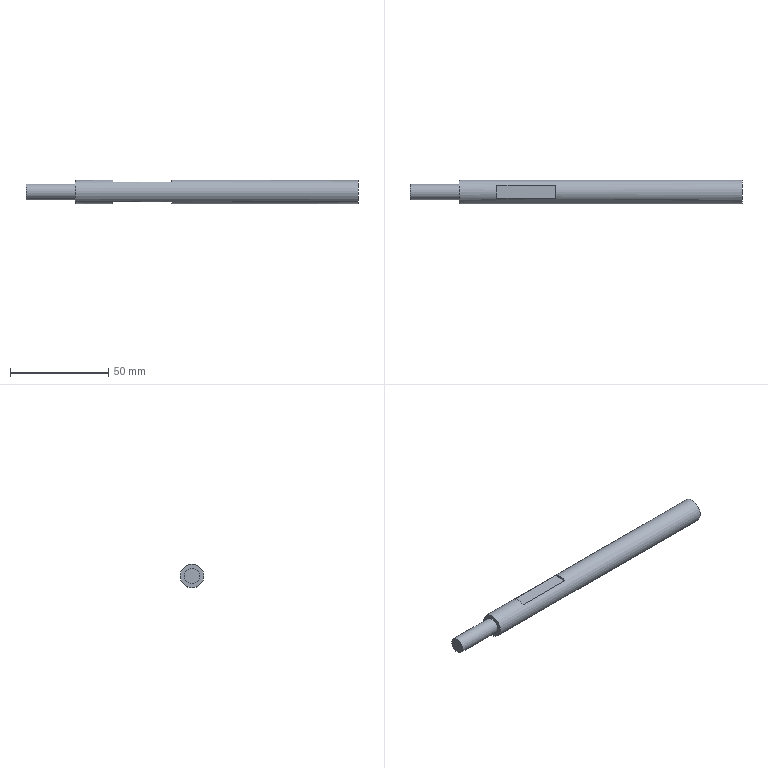Component | NX | LOCKING_SHAFT | 1 solid | 11 faces | box 169 x 12 x 12 mm | volume 17273 mm3 | plane 9 | cylinder 2 | commonest cylinder face diameters 12 x1 8 x1
STEP:
#1=CARTESIAN_POINT('',(0.,0.,0.));
#2=DIRECTION('',(0.,0.,1.));
#3=DIRECTION('',(1.,0.,0.));
#4=AXIS2_PLACEMENT_3D('',#1,#2,#3);
#5=CARTESIAN_POINT('',(-23.708,70.304,196.845));
#6=VERTEX_POINT('',#5);
#7=CARTESIAN_POINT('',(-23.708,76.937,196.845));
#8=VERTEX_POINT('',#7);
#9=CARTESIAN_POINT('',(-23.708,73.621,201.845));
#10=DIRECTION('',(1.,0.,0.));
#11=DIRECTION('',(0.,0.,1.));
#12=AXIS2_PLACEMENT_3D('',#9,#10,#11);
#13=CIRCLE('',#12,6.);
#14=CARTESIAN_POINT('',(-23.708,73.621,201.845));
#15=DIRECTION('',(-1.,0.,0.));
#16=DIRECTION('',(0.,0.,1.));
#17=AXIS2_PLACEMENT_3D('',#14,#15,#16);
#18=PLANE('',#17);
#19=CARTESIAN_POINT('',(6.,0.));
#20=CARTESIAN_POINT('',(6.,-10.392));
#21=CARTESIAN_POINT('',(-3.,-5.196));
#22=CARTESIAN_POINT('',(-12.,-0.));
#23=CARTESIAN_POINT('',(-3.,5.196));
#24=CARTESIAN_POINT('',(6.,10.392));
#25=CARTESIAN_POINT('',(6.,0.));
#26=(BOUNDED_CURVE()B_SPLINE_CURVE(2,(#19,#20,#21,#22,#23,#24,#25),.UNSPECIFIED.,.T.,.F.)B_SPLINE_CURVE_WITH_KNOTS((1,2,2,2,2,1),(-2.094,0.,2.094,4.189,6.283,8.378),.UNSPECIFIED.)CURVE()GEOMETRIC_REPRESENTATION_ITEM()RATIONAL_B_SPLINE_CURVE((1.,0.5,1.,0.5,1.,0.5,1.))REPRESENTATION_ITEM(''));
#27=(GEOMETRIC_REPRESENTATION_CONTEXT(2)PARAMETRIC_REPRESENTATION_CONTEXT()REPRESENTATION_CONTEXT('',''));
#28=DEFINITIONAL_REPRESENTATION('',(#26),#27);
#29=PCURVE('',#18,#28);
#30=CARTESIAN_POINT('',(71.092,73.621,201.845));
#31=DIRECTION('',(-1.,0.,0.));
#32=DIRECTION('',(0.,0.,1.));
#33=AXIS2_PLACEMENT_3D('',#30,#31,#32);
#34=CYLINDRICAL_SURFACE('',#33,6.);
#35=CARTESIAN_POINT('',(6.283,94.8));
#36=DIRECTION('',(-1.,0.));
#37=VECTOR('',#36,1.);
#38=LINE('',#35,#37);
#39=(GEOMETRIC_REPRESENTATION_CONTEXT(2)PARAMETRIC_REPRESENTATION_CONTEXT()REPRESENTATION_CONTEXT('',''));
#40=DEFINITIONAL_REPRESENTATION('',(#38),#39);
#41=PCURVE('',#34,#40);
#42=SURFACE_CURVE('',#13,(#29,#41),.PCURVE_S1.);
#43=EDGE_CURVE('',#6,#8,#42,.T.);
#44=ORIENTED_EDGE('',*,*,#43,.F.);
#45=CARTESIAN_POINT('',(-23.708,73.621,196.845));
#46=DIRECTION('',(0.,1.,0.));
#47=VECTOR('',#46,1.);
#48=LINE('',#45,#47);
#49=CARTESIAN_POINT('',(-5.,0.));
#50=DIRECTION('',(0.,1.));
#51=VECTOR('',#50,1.);
#52=LINE('',#49,#51);
#53=(GEOMETRIC_REPRESENTATION_CONTEXT(2)PARAMETRIC_REPRESENTATION_CONTEXT()REPRESENTATION_CONTEXT('',''));
#54=DEFINITIONAL_REPRESENTATION('',(#52),#53);
#55=PCURVE('',#18,#54);
#56=CARTESIAN_POINT('',(71.092,73.621,196.845));
#57=DIRECTION('',(0.,0.,-1.));
#58=DIRECTION('',(-1.,0.,0.));
#59=AXIS2_PLACEMENT_3D('',#56,#57,#58);
#60=PLANE('',#59);
#61=CARTESIAN_POINT('',(94.8,0.));
#62=DIRECTION('',(0.,1.));
#63=VECTOR('',#62,1.);
#64=LINE('',#61,#63);
#65=(GEOMETRIC_REPRESENTATION_CONTEXT(2)PARAMETRIC_REPRESENTATION_CONTEXT()REPRESENTATION_CONTEXT('',''));
#66=DEFINITIONAL_REPRESENTATION('',(#64),#65);
#67=PCURVE('',#60,#66);
#68=SURFACE_CURVE('',#48,(#55,#67),.PCURVE_S1.);
#69=EDGE_CURVE('',#6,#8,#68,.T.);
#70=ORIENTED_EDGE('',*,*,#69,.T.);
#71=EDGE_LOOP('',(#44,#70));
#72=FACE_BOUND('',#71,.T.);
#73=ADVANCED_FACE('',(#72),#18,.T.);
#74=CARTESIAN_POINT('',(-23.708,76.937,206.845));
#75=VERTEX_POINT('',#74);
#76=CARTESIAN_POINT('',(-23.708,73.621,207.845));
#77=VERTEX_POINT('',#76);
#78=CARTESIAN_POINT('',(-23.708,73.621,201.845));
#79=DIRECTION('',(1.,0.,0.));
#80=DIRECTION('',(0.,0.,1.));
#81=AXIS2_PLACEMENT_3D('',#78,#79,#80);
#82=CIRCLE('',#81,6.);
#83=CARTESIAN_POINT('',(-23.708,73.621,201.845));
#84=DIRECTION('',(-1.,0.,0.));
#85=DIRECTION('',(0.,0.,1.));
#86=AXIS2_PLACEMENT_3D('',#83,#84,#85);
#87=PLANE('',#86);
#88=CARTESIAN_POINT('',(6.,0.));
#89=CARTESIAN_POINT('',(6.,-10.392));
#90=CARTESIAN_POINT('',(-3.,-5.196));
#91=CARTESIAN_POINT('',(-12.,-0.));
#92=CARTESIAN_POINT('',(-3.,5.196));
#93=CARTESIAN_POINT('',(6.,10.392));
#94=CARTESIAN_POINT('',(6.,0.));
#95=(BOUNDED_CURVE()B_SPLINE_CURVE(2,(#88,#89,#90,#91,#92,#93,#94),.UNSPECIFIED.,.T.,.F.)B_SPLINE_CURVE_WITH_KNOTS((1,2,2,2,2,1),(-2.094,0.,2.094,4.189,6.283,8.378),.UNSPECIFIED.)CURVE()GEOMETRIC_REPRESENTATION_ITEM()RATIONAL_B_SPLINE_CURVE((1.,0.5,1.,0.5,1.,0.5,1.))REPRESENTATION_ITEM(''));
#96=(GEOMETRIC_REPRESENTATION_CONTEXT(2)PARAMETRIC_REPRESENTATION_CONTEXT()REPRESENTATION_CONTEXT('',''));
#97=DEFINITIONAL_REPRESENTATION('',(#95),#96);
#98=PCURVE('',#87,#97);
#99=CARTESIAN_POINT('',(6.283,94.8));
#100=DIRECTION('',(-1.,0.));
#101=VECTOR('',#100,1.);
#102=LINE('',#99,#101);
#103=(GEOMETRIC_REPRESENTATION_CONTEXT(2)PARAMETRIC_REPRESENTATION_CONTEXT()REPRESENTATION_CONTEXT('',''));
#104=DEFINITIONAL_REPRESENTATION('',(#102),#103);
#105=PCURVE('',#34,#104);
#106=SURFACE_CURVE('',#82,(#98,#105),.PCURVE_S1.);
#107=EDGE_CURVE('',#75,#77,#106,.T.);
#108=ORIENTED_EDGE('',*,*,#107,.F.);
#109=CARTESIAN_POINT('',(-23.708,70.304,206.845));
#110=VERTEX_POINT('',#109);
#111=CARTESIAN_POINT('',(-23.708,73.621,206.845));
#112=DIRECTION('',(0.,-1.,0.));
#113=VECTOR('',#112,1.);
#114=LINE('',#111,#113);
#115=CARTESIAN_POINT('',(5.,0.));
#116=DIRECTION('',(0.,-1.));
#117=VECTOR('',#116,1.);
#118=LINE('',#115,#117);
#119=(GEOMETRIC_REPRESENTATION_CONTEXT(2)PARAMETRIC_REPRESENTATION_CONTEXT()REPRESENTATION_CONTEXT('',''));
#120=DEFINITIONAL_REPRESENTATION('',(#118),#119);
#121=PCURVE('',#87,#120);
#122=CARTESIAN_POINT('',(71.092,73.621,206.845));
#123=DIRECTION('',(0.,0.,1.));
#124=DIRECTION('',(1.,0.,0.));
#125=AXIS2_PLACEMENT_3D('',#122,#123,#124);
#126=PLANE('',#125);
#127=CARTESIAN_POINT('',(-94.8,0.));
#128=DIRECTION('',(0.,-1.));
#129=VECTOR('',#128,1.);
#130=LINE('',#127,#129);
#131=(GEOMETRIC_REPRESENTATION_CONTEXT(2)PARAMETRIC_REPRESENTATION_CONTEXT()REPRESENTATION_CONTEXT('',''));
#132=DEFINITIONAL_REPRESENTATION('',(#130),#131);
#133=PCURVE('',#126,#132);
#134=SURFACE_CURVE('',#114,(#121,#133),.PCURVE_S1.);
#135=EDGE_CURVE('',#75,#110,#134,.T.);
#136=ORIENTED_EDGE('',*,*,#135,.T.);
#137=CARTESIAN_POINT('',(-23.708,73.621,201.845));
#138=DIRECTION('',(1.,0.,0.));
#139=DIRECTION('',(0.,0.,1.));
#140=AXIS2_PLACEMENT_3D('',#137,#138,#139);
#141=CIRCLE('',#140,6.);
#142=CARTESIAN_POINT('',(6.,0.));
#143=CARTESIAN_POINT('',(6.,-10.392));
#144=CARTESIAN_POINT('',(-3.,-5.196));
#145=CARTESIAN_POINT('',(-12.,-0.));
#146=CARTESIAN_POINT('',(-3.,5.196));
#147=CARTESIAN_POINT('',(6.,10.392));
#148=CARTESIAN_POINT('',(6.,0.));
#149=(BOUNDED_CURVE()B_SPLINE_CURVE(2,(#142,#143,#144,#145,#146,#147,#148),.UNSPECIFIED.,.T.,.F.)B_SPLINE_CURVE_WITH_KNOTS((1,2,2,2,2,1),(-2.094,0.,2.094,4.189,6.283,8.378),.UNSPECIFIED.)CURVE()GEOMETRIC_REPRESENTATION_ITEM()RATIONAL_B_SPLINE_CURVE((1.,0.5,1.,0.5,1.,0.5,1.))REPRESENTATION_ITEM(''));
#150=(GEOMETRIC_REPRESENTATION_CONTEXT(2)PARAMETRIC_REPRESENTATION_CONTEXT()REPRESENTATION_CONTEXT('',''));
#151=DEFINITIONAL_REPRESENTATION('',(#149),#150);
#152=PCURVE('',#87,#151);
#153=CARTESIAN_POINT('',(12.566,94.8));
#154=DIRECTION('',(-1.,0.));
#155=VECTOR('',#154,1.);
#156=LINE('',#153,#155);
#157=(GEOMETRIC_REPRESENTATION_CONTEXT(2)PARAMETRIC_REPRESENTATION_CONTEXT()REPRESENTATION_CONTEXT('',''));
#158=DEFINITIONAL_REPRESENTATION('',(#156),#157);
#159=PCURVE('',#34,#158);
#160=SURFACE_CURVE('',#141,(#152,#159),.PCURVE_S1.);
#161=EDGE_CURVE('',#77,#110,#160,.T.);
#162=ORIENTED_EDGE('',*,*,#161,.F.);
#163=EDGE_LOOP('',(#108,#136,#162));
#164=FACE_BOUND('',#163,.T.);
#165=ADVANCED_FACE('',(#164),#87,.T.);
#166=CARTESIAN_POINT('',(71.092,73.621,207.845));
#167=VERTEX_POINT('',#166);
#168=CARTESIAN_POINT('',(71.092,73.621,201.845));
#169=DIRECTION('',(-1.,0.,0.));
#170=DIRECTION('',(0.,0.,1.));
#171=AXIS2_PLACEMENT_3D('',#168,#169,#170);
#172=CIRCLE('',#171,6.);
#173=CARTESIAN_POINT('',(71.092,73.621,201.845));
#174=DIRECTION('',(1.,0.,0.));
#175=DIRECTION('',(0.,0.,-1.));
#176=AXIS2_PLACEMENT_3D('',#173,#174,#175);
#177=PLANE('',#176);
#178=CARTESIAN_POINT('',(-6.,0.));
#179=CARTESIAN_POINT('',(-6.,10.392));
#180=CARTESIAN_POINT('',(3.,5.196));
#181=CARTESIAN_POINT('',(12.,0.));
#182=CARTESIAN_POINT('',(3.,-5.196));
#183=CARTESIAN_POINT('',(-6.,-10.392));
#184=CARTESIAN_POINT('',(-6.,0.));
#185=(BOUNDED_CURVE()B_SPLINE_CURVE(2,(#178,#179,#180,#181,#182,#183,#184),.UNSPECIFIED.,.T.,.F.)B_SPLINE_CURVE_WITH_KNOTS((1,2,2,2,2,1),(-2.094,0.,2.094,4.189,6.283,8.378),.UNSPECIFIED.)CURVE()GEOMETRIC_REPRESENTATION_ITEM()RATIONAL_B_SPLINE_CURVE((1.,0.5,1.,0.5,1.,0.5,1.))REPRESENTATION_ITEM(''));
#186=(GEOMETRIC_REPRESENTATION_CONTEXT(2)PARAMETRIC_REPRESENTATION_CONTEXT()REPRESENTATION_CONTEXT('',''));
#187=DEFINITIONAL_REPRESENTATION('',(#185),#186);
#188=PCURVE('',#177,#187);
#189=CARTESIAN_POINT('',(0.,0.));
#190=DIRECTION('',(1.,0.));
#191=VECTOR('',#190,1.);
#192=LINE('',#189,#191);
#193=(GEOMETRIC_REPRESENTATION_CONTEXT(2)PARAMETRIC_REPRESENTATION_CONTEXT()REPRESENTATION_CONTEXT('',''));
#194=DEFINITIONAL_REPRESENTATION('',(#192),#193);
#195=PCURVE('',#34,#194);
#196=SURFACE_CURVE('',#172,(#188,#195),.PCURVE_S1.);
#197=EDGE_CURVE('',#167,#167,#196,.T.);
#198=ORIENTED_EDGE('',*,*,#197,.F.);
#199=EDGE_LOOP('',(#198));
#200=FACE_BOUND('',#199,.T.);
#201=ADVANCED_FACE('',(#200),#177,.T.);
#202=ORIENTED_EDGE('',*,*,#107,.T.);
#203=CARTESIAN_POINT('',(71.092,73.621,207.845));
#204=CARTESIAN_POINT('',(-23.708,73.621,207.845));
#205=B_SPLINE_CURVE_WITH_KNOTS('',1,(#203,#204),.UNSPECIFIED.,.F.,.F.,(2,2),(0.,94.8),.PIECEWISE_BEZIER_KNOTS.);
#206=CARTESIAN_POINT('',(0.,0.));
#207=DIRECTION('',(0.,1.));
#208=VECTOR('',#207,1.);
#209=LINE('',#206,#208);
#210=(GEOMETRIC_REPRESENTATION_CONTEXT(2)PARAMETRIC_REPRESENTATION_CONTEXT()REPRESENTATION_CONTEXT('',''));
#211=DEFINITIONAL_REPRESENTATION('',(#209),#210);
#212=PCURVE('',#34,#211);
#213=CARTESIAN_POINT('',(6.283,0.));
#214=DIRECTION('',(0.,1.));
#215=VECTOR('',#214,1.);
#216=LINE('',#213,#215);
#217=(GEOMETRIC_REPRESENTATION_CONTEXT(2)PARAMETRIC_REPRESENTATION_CONTEXT()REPRESENTATION_CONTEXT('',''));
#218=DEFINITIONAL_REPRESENTATION('',(#216),#217);
#219=PCURVE('',#34,#218);
#220=SEAM_CURVE('',#205,(#212,#219),.PCURVE_S1.);
#221=EDGE_CURVE('',#167,#77,#220,.T.);
#222=ORIENTED_EDGE('',*,*,#221,.F.);
#223=ORIENTED_EDGE('',*,*,#197,.T.);
#224=ORIENTED_EDGE('',*,*,#221,.T.);
#225=ORIENTED_EDGE('',*,*,#161,.T.);
#226=CARTESIAN_POINT('',(-53.708,70.304,206.845));
#227=VERTEX_POINT('',#226);
#228=CARTESIAN_POINT('',(-23.708,70.304,206.845));
#229=DIRECTION('',(-1.,0.,0.));
#230=VECTOR('',#229,1.);
#231=LINE('',#228,#230);
#232=CARTESIAN_POINT('',(5.697,94.8));
#233=DIRECTION('',(0.,1.));
#234=VECTOR('',#233,1.);
#235=LINE('',#232,#234);
#236=(GEOMETRIC_REPRESENTATION_CONTEXT(2)PARAMETRIC_REPRESENTATION_CONTEXT()REPRESENTATION_CONTEXT('',''));
#237=DEFINITIONAL_REPRESENTATION('',(#235),#236);
#238=PCURVE('',#34,#237);
#239=CARTESIAN_POINT('',(-94.8,-3.317));
#240=DIRECTION('',(-1.,0.));
#241=VECTOR('',#240,1.);
#242=LINE('',#239,#241);
#243=(GEOMETRIC_REPRESENTATION_CONTEXT(2)PARAMETRIC_REPRESENTATION_CONTEXT()REPRESENTATION_CONTEXT('',''));
#244=DEFINITIONAL_REPRESENTATION('',(#242),#243);
#245=PCURVE('',#126,#244);
#246=SURFACE_CURVE('',#231,(#238,#245),.PCURVE_S1.);
#247=EDGE_CURVE('',#110,#227,#246,.T.);
#248=ORIENTED_EDGE('',*,*,#247,.T.);
#249=CARTESIAN_POINT('',(-53.708,73.621,207.845));
#250=VERTEX_POINT('',#249);
#251=CARTESIAN_POINT('',(-53.708,73.621,201.845));
#252=DIRECTION('',(-1.,0.,0.));
#253=DIRECTION('',(0.,0.,1.));
#254=AXIS2_PLACEMENT_3D('',#251,#252,#253);
#255=CIRCLE('',#254,6.);
#256=CARTESIAN_POINT('',(0.,124.8));
#257=DIRECTION('',(1.,0.));
#258=VECTOR('',#257,1.);
#259=LINE('',#256,#258);
#260=(GEOMETRIC_REPRESENTATION_CONTEXT(2)PARAMETRIC_REPRESENTATION_CONTEXT()REPRESENTATION_CONTEXT('',''));
#261=DEFINITIONAL_REPRESENTATION('',(#259),#260);
#262=PCURVE('',#34,#261);
#263=CARTESIAN_POINT('',(-53.708,73.621,201.845));
#264=DIRECTION('',(1.,0.,0.));
#265=DIRECTION('',(0.,0.,-1.));
#266=AXIS2_PLACEMENT_3D('',#263,#264,#265);
#267=PLANE('',#266);
#268=CARTESIAN_POINT('',(-6.,0.));
#269=CARTESIAN_POINT('',(-6.,10.392));
#270=CARTESIAN_POINT('',(3.,5.196));
#271=CARTESIAN_POINT('',(12.,0.));
#272=CARTESIAN_POINT('',(3.,-5.196));
#273=CARTESIAN_POINT('',(-6.,-10.392));
#274=CARTESIAN_POINT('',(-6.,0.));
#275=(BOUNDED_CURVE()B_SPLINE_CURVE(2,(#268,#269,#270,#271,#272,#273,#274),.UNSPECIFIED.,.T.,.F.)B_SPLINE_CURVE_WITH_KNOTS((1,2,2,2,2,1),(-2.094,0.,2.094,4.189,6.283,8.378),.UNSPECIFIED.)CURVE()GEOMETRIC_REPRESENTATION_ITEM()RATIONAL_B_SPLINE_CURVE((1.,0.5,1.,0.5,1.,0.5,1.))REPRESENTATION_ITEM(''));
#276=(GEOMETRIC_REPRESENTATION_CONTEXT(2)PARAMETRIC_REPRESENTATION_CONTEXT()REPRESENTATION_CONTEXT('',''));
#277=DEFINITIONAL_REPRESENTATION('',(#275),#276);
#278=PCURVE('',#267,#277);
#279=SURFACE_CURVE('',#255,(#262,#278),.PCURVE_S1.);
#280=EDGE_CURVE('',#227,#250,#279,.T.);
#281=ORIENTED_EDGE('',*,*,#280,.T.);
#282=CARTESIAN_POINT('',(-72.908,73.621,207.845));
#283=VERTEX_POINT('',#282);
#284=CARTESIAN_POINT('',(-53.708,73.621,207.845));
#285=CARTESIAN_POINT('',(-72.908,73.621,207.845));
#286=B_SPLINE_CURVE_WITH_KNOTS('',1,(#284,#285),.UNSPECIFIED.,.F.,.F.,(2,2),(124.8,144.),.PIECEWISE_BEZIER_KNOTS.);
#287=CARTESIAN_POINT('',(6.283,0.));
#288=DIRECTION('',(0.,1.));
#289=VECTOR('',#288,1.);
#290=LINE('',#287,#289);
#291=(GEOMETRIC_REPRESENTATION_CONTEXT(2)PARAMETRIC_REPRESENTATION_CONTEXT()REPRESENTATION_CONTEXT('',''));
#292=DEFINITIONAL_REPRESENTATION('',(#290),#291);
#293=PCURVE('',#34,#292);
#294=CARTESIAN_POINT('',(0.,0.));
#295=DIRECTION('',(0.,1.));
#296=VECTOR('',#295,1.);
#297=LINE('',#294,#296);
#298=(GEOMETRIC_REPRESENTATION_CONTEXT(2)PARAMETRIC_REPRESENTATION_CONTEXT()REPRESENTATION_CONTEXT('',''));
#299=DEFINITIONAL_REPRESENTATION('',(#297),#298);
#300=PCURVE('',#34,#299);
#301=SEAM_CURVE('',#286,(#293,#300),.PCURVE_S1.);
#302=EDGE_CURVE('',#250,#283,#301,.T.);
#303=ORIENTED_EDGE('',*,*,#302,.T.);
#304=CARTESIAN_POINT('',(-72.908,73.621,201.845));
#305=DIRECTION('',(1.,0.,0.));
#306=DIRECTION('',(0.,0.,1.));
#307=AXIS2_PLACEMENT_3D('',#304,#305,#306);
#308=CIRCLE('',#307,6.);
#309=CARTESIAN_POINT('',(6.283,144.));
#310=DIRECTION('',(-1.,0.));
#311=VECTOR('',#310,1.);
#312=LINE('',#309,#311);
#313=(GEOMETRIC_REPRESENTATION_CONTEXT(2)PARAMETRIC_REPRESENTATION_CONTEXT()REPRESENTATION_CONTEXT('',''));
#314=DEFINITIONAL_REPRESENTATION('',(#312),#313);
#315=PCURVE('',#34,#314);
#316=CARTESIAN_POINT('',(-72.908,73.621,201.845));
#317=DIRECTION('',(-1.,0.,0.));
#318=DIRECTION('',(0.,0.,1.));
#319=AXIS2_PLACEMENT_3D('',#316,#317,#318);
#320=PLANE('',#319);
#321=CARTESIAN_POINT('',(6.,0.));
#322=CARTESIAN_POINT('',(6.,-10.392));
#323=CARTESIAN_POINT('',(-3.,-5.196));
#324=CARTESIAN_POINT('',(-12.,-0.));
#325=CARTESIAN_POINT('',(-3.,5.196));
#326=CARTESIAN_POINT('',(6.,10.392));
#327=CARTESIAN_POINT('',(6.,0.));
#328=(BOUNDED_CURVE()B_SPLINE_CURVE(2,(#321,#322,#323,#324,#325,#326,#327),.UNSPECIFIED.,.T.,.F.)B_SPLINE_CURVE_WITH_KNOTS((1,2,2,2,2,1),(-2.094,0.,2.094,4.189,6.283,8.378),.UNSPECIFIED.)CURVE()GEOMETRIC_REPRESENTATION_ITEM()RATIONAL_B_SPLINE_CURVE((1.,0.5,1.,0.5,1.,0.5,1.))REPRESENTATION_ITEM(''));
#329=(GEOMETRIC_REPRESENTATION_CONTEXT(2)PARAMETRIC_REPRESENTATION_CONTEXT()REPRESENTATION_CONTEXT('',''));
#330=DEFINITIONAL_REPRESENTATION('',(#328),#329);
#331=PCURVE('',#320,#330);
#332=SURFACE_CURVE('',#308,(#315,#331),.PCURVE_S1.);
#333=EDGE_CURVE('',#283,#283,#332,.T.);
#334=ORIENTED_EDGE('',*,*,#333,.T.);
#335=ORIENTED_EDGE('',*,*,#302,.F.);
#336=CARTESIAN_POINT('',(-53.708,76.937,206.845));
#337=VERTEX_POINT('',#336);
#338=CARTESIAN_POINT('',(-53.708,73.621,201.845));
#339=DIRECTION('',(-1.,0.,0.));
#340=DIRECTION('',(0.,0.,1.));
#341=AXIS2_PLACEMENT_3D('',#338,#339,#340);
#342=CIRCLE('',#341,6.);
#343=CARTESIAN_POINT('',(-6.283,124.8));
#344=DIRECTION('',(1.,0.));
#345=VECTOR('',#344,1.);
#346=LINE('',#343,#345);
#347=(GEOMETRIC_REPRESENTATION_CONTEXT(2)PARAMETRIC_REPRESENTATION_CONTEXT()REPRESENTATION_CONTEXT('',''));
#348=DEFINITIONAL_REPRESENTATION('',(#346),#347);
#349=PCURVE('',#34,#348);
#350=CARTESIAN_POINT('',(-6.,0.));
#351=CARTESIAN_POINT('',(-6.,10.392));
#352=CARTESIAN_POINT('',(3.,5.196));
#353=CARTESIAN_POINT('',(12.,0.));
#354=CARTESIAN_POINT('',(3.,-5.196));
#355=CARTESIAN_POINT('',(-6.,-10.392));
#356=CARTESIAN_POINT('',(-6.,0.));
#357=(BOUNDED_CURVE()B_SPLINE_CURVE(2,(#350,#351,#352,#353,#354,#355,#356),.UNSPECIFIED.,.T.,.F.)B_SPLINE_CURVE_WITH_KNOTS((1,2,2,2,2,1),(-2.094,0.,2.094,4.189,6.283,8.378),.UNSPECIFIED.)CURVE()GEOMETRIC_REPRESENTATION_ITEM()RATIONAL_B_SPLINE_CURVE((1.,0.5,1.,0.5,1.,0.5,1.))REPRESENTATION_ITEM(''));
#358=(GEOMETRIC_REPRESENTATION_CONTEXT(2)PARAMETRIC_REPRESENTATION_CONTEXT()REPRESENTATION_CONTEXT('',''));
#359=DEFINITIONAL_REPRESENTATION('',(#357),#358);
#360=PCURVE('',#267,#359);
#361=SURFACE_CURVE('',#342,(#349,#360),.PCURVE_S1.);
#362=EDGE_CURVE('',#250,#337,#361,.T.);
#363=ORIENTED_EDGE('',*,*,#362,.T.);
#364=CARTESIAN_POINT('',(-23.708,76.937,206.845));
#365=DIRECTION('',(1.,0.,0.));
#366=VECTOR('',#365,1.);
#367=LINE('',#364,#366);
#368=CARTESIAN_POINT('',(0.5857,94.8));
#369=DIRECTION('',(0.,-1.));
#370=VECTOR('',#369,1.);
#371=LINE('',#368,#370);
#372=(GEOMETRIC_REPRESENTATION_CONTEXT(2)PARAMETRIC_REPRESENTATION_CONTEXT()REPRESENTATION_CONTEXT('',''));
#373=DEFINITIONAL_REPRESENTATION('',(#371),#372);
#374=PCURVE('',#34,#373);
#375=CARTESIAN_POINT('',(-94.8,3.317));
#376=DIRECTION('',(1.,0.));
#377=VECTOR('',#376,1.);
#378=LINE('',#375,#377);
#379=(GEOMETRIC_REPRESENTATION_CONTEXT(2)PARAMETRIC_REPRESENTATION_CONTEXT()REPRESENTATION_CONTEXT('',''));
#380=DEFINITIONAL_REPRESENTATION('',(#378),#379);
#381=PCURVE('',#126,#380);
#382=SURFACE_CURVE('',#367,(#374,#381),.PCURVE_S1.);
#383=EDGE_CURVE('',#337,#75,#382,.T.);
#384=ORIENTED_EDGE('',*,*,#383,.T.);
#385=EDGE_LOOP('',(#202,#222,#223,#224,#225,#248,#281,#303,#334,#335,#363,#384));
#386=FACE_BOUND('',#385,.T.);
#387=CARTESIAN_POINT('',(-53.708,70.304,196.845));
#388=VERTEX_POINT('',#387);
#389=CARTESIAN_POINT('',(-23.708,70.304,196.845));
#390=DIRECTION('',(1.,0.,0.));
#391=VECTOR('',#390,1.);
#392=LINE('',#389,#391);
#393=CARTESIAN_POINT('',(3.727,94.8));
#394=DIRECTION('',(0.,-1.));
#395=VECTOR('',#394,1.);
#396=LINE('',#393,#395);
#397=(GEOMETRIC_REPRESENTATION_CONTEXT(2)PARAMETRIC_REPRESENTATION_CONTEXT()REPRESENTATION_CONTEXT('',''));
#398=DEFINITIONAL_REPRESENTATION('',(#396),#397);
#399=PCURVE('',#34,#398);
#400=CARTESIAN_POINT('',(94.8,-3.317));
#401=DIRECTION('',(-1.,0.));
#402=VECTOR('',#401,1.);
#403=LINE('',#400,#402);
#404=(GEOMETRIC_REPRESENTATION_CONTEXT(2)PARAMETRIC_REPRESENTATION_CONTEXT()REPRESENTATION_CONTEXT('',''));
#405=DEFINITIONAL_REPRESENTATION('',(#403),#404);
#406=PCURVE('',#60,#405);
#407=SURFACE_CURVE('',#392,(#399,#406),.PCURVE_S1.);
#408=EDGE_CURVE('',#388,#6,#407,.T.);
#409=ORIENTED_EDGE('',*,*,#408,.T.);
#410=ORIENTED_EDGE('',*,*,#43,.T.);
#411=CARTESIAN_POINT('',(-53.708,76.937,196.845));
#412=VERTEX_POINT('',#411);
#413=CARTESIAN_POINT('',(-23.708,76.937,196.845));
#414=DIRECTION('',(-1.,0.,0.));
#415=VECTOR('',#414,1.);
#416=LINE('',#413,#415);
#417=CARTESIAN_POINT('',(2.556,94.8));
#418=DIRECTION('',(0.,1.));
#419=VECTOR('',#418,1.);
#420=LINE('',#417,#419);
#421=(GEOMETRIC_REPRESENTATION_CONTEXT(2)PARAMETRIC_REPRESENTATION_CONTEXT()REPRESENTATION_CONTEXT('',''));
#422=DEFINITIONAL_REPRESENTATION('',(#420),#421);
#423=PCURVE('',#34,#422);
#424=CARTESIAN_POINT('',(94.8,3.317));
#425=DIRECTION('',(1.,0.));
#426=VECTOR('',#425,1.);
#427=LINE('',#424,#426);
#428=(GEOMETRIC_REPRESENTATION_CONTEXT(2)PARAMETRIC_REPRESENTATION_CONTEXT()REPRESENTATION_CONTEXT('',''));
#429=DEFINITIONAL_REPRESENTATION('',(#427),#428);
#430=PCURVE('',#60,#429);
#431=SURFACE_CURVE('',#416,(#423,#430),.PCURVE_S1.);
#432=EDGE_CURVE('',#8,#412,#431,.T.);
#433=ORIENTED_EDGE('',*,*,#432,.T.);
#434=CARTESIAN_POINT('',(-53.708,73.621,201.845));
#435=DIRECTION('',(-1.,0.,0.));
#436=DIRECTION('',(0.,0.,1.));
#437=AXIS2_PLACEMENT_3D('',#434,#435,#436);
#438=CIRCLE('',#437,6.);
#439=CARTESIAN_POINT('',(0.,124.8));
#440=DIRECTION('',(1.,0.));
#441=VECTOR('',#440,1.);
#442=LINE('',#439,#441);
#443=(GEOMETRIC_REPRESENTATION_CONTEXT(2)PARAMETRIC_REPRESENTATION_CONTEXT()REPRESENTATION_CONTEXT('',''));
#444=DEFINITIONAL_REPRESENTATION('',(#442),#443);
#445=PCURVE('',#34,#444);
#446=CARTESIAN_POINT('',(-53.708,73.621,201.845));
#447=DIRECTION('',(1.,0.,0.));
#448=DIRECTION('',(0.,0.,-1.));
#449=AXIS2_PLACEMENT_3D('',#446,#447,#448);
#450=PLANE('',#449);
#451=CARTESIAN_POINT('',(-6.,0.));
#452=CARTESIAN_POINT('',(-6.,10.392));
#453=CARTESIAN_POINT('',(3.,5.196));
#454=CARTESIAN_POINT('',(12.,0.));
#455=CARTESIAN_POINT('',(3.,-5.196));
#456=CARTESIAN_POINT('',(-6.,-10.392));
#457=CARTESIAN_POINT('',(-6.,0.));
#458=(BOUNDED_CURVE()B_SPLINE_CURVE(2,(#451,#452,#453,#454,#455,#456,#457),.UNSPECIFIED.,.T.,.F.)B_SPLINE_CURVE_WITH_KNOTS((1,2,2,2,2,1),(-2.094,0.,2.094,4.189,6.283,8.378),.UNSPECIFIED.)CURVE()GEOMETRIC_REPRESENTATION_ITEM()RATIONAL_B_SPLINE_CURVE((1.,0.5,1.,0.5,1.,0.5,1.))REPRESENTATION_ITEM(''));
#459=(GEOMETRIC_REPRESENTATION_CONTEXT(2)PARAMETRIC_REPRESENTATION_CONTEXT()REPRESENTATION_CONTEXT('',''));
#460=DEFINITIONAL_REPRESENTATION('',(#458),#459);
#461=PCURVE('',#450,#460);
#462=SURFACE_CURVE('',#438,(#445,#461),.PCURVE_S1.);
#463=EDGE_CURVE('',#412,#388,#462,.T.);
#464=ORIENTED_EDGE('',*,*,#463,.T.);
#465=EDGE_LOOP('',(#409,#410,#433,#464));
#466=FACE_BOUND('',#465,.T.);
#467=ADVANCED_FACE('',(#386,#466),#34,.T.);
#468=ORIENTED_EDGE('',*,*,#383,.F.);
#469=CARTESIAN_POINT('',(-53.708,73.621,206.845));
#470=DIRECTION('',(0.,1.,0.));
#471=VECTOR('',#470,1.);
#472=LINE('',#469,#471);
#473=CARTESIAN_POINT('',(-124.8,0.));
#474=DIRECTION('',(0.,1.));
#475=VECTOR('',#474,1.);
#476=LINE('',#473,#475);
#477=(GEOMETRIC_REPRESENTATION_CONTEXT(2)PARAMETRIC_REPRESENTATION_CONTEXT()REPRESENTATION_CONTEXT('',''));
#478=DEFINITIONAL_REPRESENTATION('',(#476),#477);
#479=PCURVE('',#126,#478);
#480=CARTESIAN_POINT('',(-5.,0.));
#481=DIRECTION('',(0.,1.));
#482=VECTOR('',#481,1.);
#483=LINE('',#480,#482);
#484=(GEOMETRIC_REPRESENTATION_CONTEXT(2)PARAMETRIC_REPRESENTATION_CONTEXT()REPRESENTATION_CONTEXT('',''));
#485=DEFINITIONAL_REPRESENTATION('',(#483),#484);
#486=PCURVE('',#267,#485);
#487=SURFACE_CURVE('',#472,(#479,#486),.PCURVE_S1.);
#488=EDGE_CURVE('',#227,#337,#487,.T.);
#489=ORIENTED_EDGE('',*,*,#488,.F.);
#490=ORIENTED_EDGE('',*,*,#247,.F.);
#491=ORIENTED_EDGE('',*,*,#135,.F.);
#492=EDGE_LOOP('',(#468,#489,#490,#491));
#493=FACE_BOUND('',#492,.T.);
#494=ADVANCED_FACE('',(#493),#126,.T.);
#495=ORIENTED_EDGE('',*,*,#408,.F.);
#496=CARTESIAN_POINT('',(-53.708,73.621,196.845));
#497=DIRECTION('',(0.,-1.,0.));
#498=VECTOR('',#497,1.);
#499=LINE('',#496,#498);
#500=CARTESIAN_POINT('',(124.8,0.));
#501=DIRECTION('',(0.,-1.));
#502=VECTOR('',#501,1.);
#503=LINE('',#500,#502);
#504=(GEOMETRIC_REPRESENTATION_CONTEXT(2)PARAMETRIC_REPRESENTATION_CONTEXT()REPRESENTATION_CONTEXT('',''));
#505=DEFINITIONAL_REPRESENTATION('',(#503),#504);
#506=PCURVE('',#60,#505);
#507=CARTESIAN_POINT('',(5.,0.));
#508=DIRECTION('',(0.,-1.));
#509=VECTOR('',#508,1.);
#510=LINE('',#507,#509);
#511=(GEOMETRIC_REPRESENTATION_CONTEXT(2)PARAMETRIC_REPRESENTATION_CONTEXT()REPRESENTATION_CONTEXT('',''));
#512=DEFINITIONAL_REPRESENTATION('',(#510),#511);
#513=PCURVE('',#450,#512);
#514=SURFACE_CURVE('',#499,(#506,#513),.PCURVE_S1.);
#515=EDGE_CURVE('',#412,#388,#514,.T.);
#516=ORIENTED_EDGE('',*,*,#515,.F.);
#517=ORIENTED_EDGE('',*,*,#432,.F.);
#518=ORIENTED_EDGE('',*,*,#69,.F.);
#519=EDGE_LOOP('',(#495,#516,#517,#518));
#520=FACE_BOUND('',#519,.T.);
#521=ADVANCED_FACE('',(#520),#60,.T.);
#522=ORIENTED_EDGE('',*,*,#463,.F.);
#523=ORIENTED_EDGE('',*,*,#515,.T.);
#524=EDGE_LOOP('',(#522,#523));
#525=FACE_BOUND('',#524,.T.);
#526=ADVANCED_FACE('',(#525),#450,.T.);
#527=CARTESIAN_POINT('',(-72.908,73.621,205.845));
#528=VERTEX_POINT('',#527);
#529=CARTESIAN_POINT('',(-72.908,73.621,201.845));
#530=DIRECTION('',(-1.,0.,0.));
#531=DIRECTION('',(0.,0.,1.));
#532=AXIS2_PLACEMENT_3D('',#529,#530,#531);
#533=CIRCLE('',#532,4.);
#534=CARTESIAN_POINT('',(0.,0.));
#535=DIRECTION('',(1.,0.));
#536=AXIS2_PLACEMENT_2D('',#534,#535);
#537=CIRCLE('',#536,4.);
#538=(GEOMETRIC_REPRESENTATION_CONTEXT(2)PARAMETRIC_REPRESENTATION_CONTEXT()REPRESENTATION_CONTEXT('',''));
#539=DEFINITIONAL_REPRESENTATION('',(#537),#538);
#540=PCURVE('',#320,#539);
#541=CARTESIAN_POINT('',(-72.908,73.621,201.845));
#542=DIRECTION('',(-1.,0.,0.));
#543=DIRECTION('',(0.,0.,1.));
#544=AXIS2_PLACEMENT_3D('',#541,#542,#543);
#545=CYLINDRICAL_SURFACE('',#544,4.);
#546=CARTESIAN_POINT('',(0.,0.));
#547=DIRECTION('',(1.,0.));
#548=VECTOR('',#547,1.);
#549=LINE('',#546,#548);
#550=(GEOMETRIC_REPRESENTATION_CONTEXT(2)PARAMETRIC_REPRESENTATION_CONTEXT()REPRESENTATION_CONTEXT('',''));
#551=DEFINITIONAL_REPRESENTATION('',(#549),#550);
#552=PCURVE('',#545,#551);
#553=SURFACE_CURVE('',#533,(#540,#552),.PCURVE_S1.);
#554=EDGE_CURVE('',#528,#528,#553,.T.);
#555=ORIENTED_EDGE('',*,*,#554,.F.);
#556=EDGE_LOOP('',(#555));
#557=FACE_BOUND('',#556,.T.);
#558=ORIENTED_EDGE('',*,*,#333,.F.);
#559=EDGE_LOOP('',(#558));
#560=FACE_BOUND('',#559,.T.);
#561=ADVANCED_FACE('',(#557,#560),#320,.T.);
#562=ORIENTED_EDGE('',*,*,#280,.F.);
#563=ORIENTED_EDGE('',*,*,#488,.T.);
#564=ORIENTED_EDGE('',*,*,#362,.F.);
#565=EDGE_LOOP('',(#562,#563,#564));
#566=FACE_BOUND('',#565,.T.);
#567=ADVANCED_FACE('',(#566),#267,.T.);
#568=CARTESIAN_POINT('',(-97.908,73.621,205.845));
#569=VERTEX_POINT('',#568);
#570=CARTESIAN_POINT('',(-97.908,73.621,201.845));
#571=DIRECTION('',(1.,0.,0.));
#572=DIRECTION('',(0.,0.,1.));
#573=AXIS2_PLACEMENT_3D('',#570,#571,#572);
#574=CIRCLE('',#573,4.);
#575=CARTESIAN_POINT('',(-97.908,73.621,201.845));
#576=DIRECTION('',(-1.,0.,0.));
#577=DIRECTION('',(0.,0.,1.));
#578=AXIS2_PLACEMENT_3D('',#575,#576,#577);
#579=PLANE('',#578);
#580=CARTESIAN_POINT('',(4.,0.));
#581=CARTESIAN_POINT('',(4.,-6.928));
#582=CARTESIAN_POINT('',(-2.,-3.464));
#583=CARTESIAN_POINT('',(-8.,-0.));
#584=CARTESIAN_POINT('',(-2.,3.464));
#585=CARTESIAN_POINT('',(4.,6.928));
#586=CARTESIAN_POINT('',(4.,0.));
#587=(BOUNDED_CURVE()B_SPLINE_CURVE(2,(#580,#581,#582,#583,#584,#585,#586),.UNSPECIFIED.,.T.,.F.)B_SPLINE_CURVE_WITH_KNOTS((1,2,2,2,2,1),(-2.094,0.,2.094,4.189,6.283,8.378),.UNSPECIFIED.)CURVE()GEOMETRIC_REPRESENTATION_ITEM()RATIONAL_B_SPLINE_CURVE((1.,0.5,1.,0.5,1.,0.5,1.))REPRESENTATION_ITEM(''));
#588=(GEOMETRIC_REPRESENTATION_CONTEXT(2)PARAMETRIC_REPRESENTATION_CONTEXT()REPRESENTATION_CONTEXT('',''));
#589=DEFINITIONAL_REPRESENTATION('',(#587),#588);
#590=PCURVE('',#579,#589);
#591=CARTESIAN_POINT('',(6.283,25.));
#592=DIRECTION('',(-1.,0.));
#593=VECTOR('',#592,1.);
#594=LINE('',#591,#593);
#595=(GEOMETRIC_REPRESENTATION_CONTEXT(2)PARAMETRIC_REPRESENTATION_CONTEXT()REPRESENTATION_CONTEXT('',''));
#596=DEFINITIONAL_REPRESENTATION('',(#594),#595);
#597=PCURVE('',#545,#596);
#598=SURFACE_CURVE('',#574,(#590,#597),.PCURVE_S1.);
#599=EDGE_CURVE('',#569,#569,#598,.T.);
#600=ORIENTED_EDGE('',*,*,#599,.F.);
#601=EDGE_LOOP('',(#600));
#602=FACE_BOUND('',#601,.T.);
#603=ADVANCED_FACE('',(#602),#579,.T.);
#604=ORIENTED_EDGE('',*,*,#599,.T.);
#605=CARTESIAN_POINT('',(-72.908,73.621,205.845));
#606=CARTESIAN_POINT('',(-97.908,73.621,205.845));
#607=B_SPLINE_CURVE_WITH_KNOTS('',1,(#605,#606),.UNSPECIFIED.,.F.,.F.,(2,2),(0.,25.),.PIECEWISE_BEZIER_KNOTS.);
#608=CARTESIAN_POINT('',(0.,0.));
#609=DIRECTION('',(0.,1.));
#610=VECTOR('',#609,1.);
#611=LINE('',#608,#610);
#612=(GEOMETRIC_REPRESENTATION_CONTEXT(2)PARAMETRIC_REPRESENTATION_CONTEXT()REPRESENTATION_CONTEXT('',''));
#613=DEFINITIONAL_REPRESENTATION('',(#611),#612);
#614=PCURVE('',#545,#613);
#615=CARTESIAN_POINT('',(6.283,0.));
#616=DIRECTION('',(0.,1.));
#617=VECTOR('',#616,1.);
#618=LINE('',#615,#617);
#619=(GEOMETRIC_REPRESENTATION_CONTEXT(2)PARAMETRIC_REPRESENTATION_CONTEXT()REPRESENTATION_CONTEXT('',''));
#620=DEFINITIONAL_REPRESENTATION('',(#618),#619);
#621=PCURVE('',#545,#620);
#622=SEAM_CURVE('',#607,(#614,#621),.PCURVE_S1.);
#623=EDGE_CURVE('',#528,#569,#622,.T.);
#624=ORIENTED_EDGE('',*,*,#623,.F.);
#625=ORIENTED_EDGE('',*,*,#554,.T.);
#626=ORIENTED_EDGE('',*,*,#623,.T.);
#627=EDGE_LOOP('',(#604,#624,#625,#626));
#628=FACE_BOUND('',#627,.T.);
#629=ADVANCED_FACE('',(#628),#545,.T.);
#630=CLOSED_SHELL('',(#73,#165,#201,#467,#494,#521,#526,#561,#567,#603,#629));
#631=MANIFOLD_SOLID_BREP('',#630);
#632=(LENGTH_UNIT()NAMED_UNIT(*)SI_UNIT(.MILLI.,.METRE.));
#633=UNCERTAINTY_MEASURE_WITH_UNIT(LENGTH_MEASURE(0.000002),#632,'','');
#634=(NAMED_UNIT(*)PLANE_ANGLE_UNIT()SI_UNIT($,.RADIAN.));
#635=(NAMED_UNIT(*)SI_UNIT($,.STERADIAN.)SOLID_ANGLE_UNIT());
#636=(GEOMETRIC_REPRESENTATION_CONTEXT(3)GLOBAL_UNCERTAINTY_ASSIGNED_CONTEXT((#633))GLOBAL_UNIT_ASSIGNED_CONTEXT((#632,#634,#635))REPRESENTATION_CONTEXT('',''));
#637=ADVANCED_BREP_SHAPE_REPRESENTATION('',(#4,#631),#636);